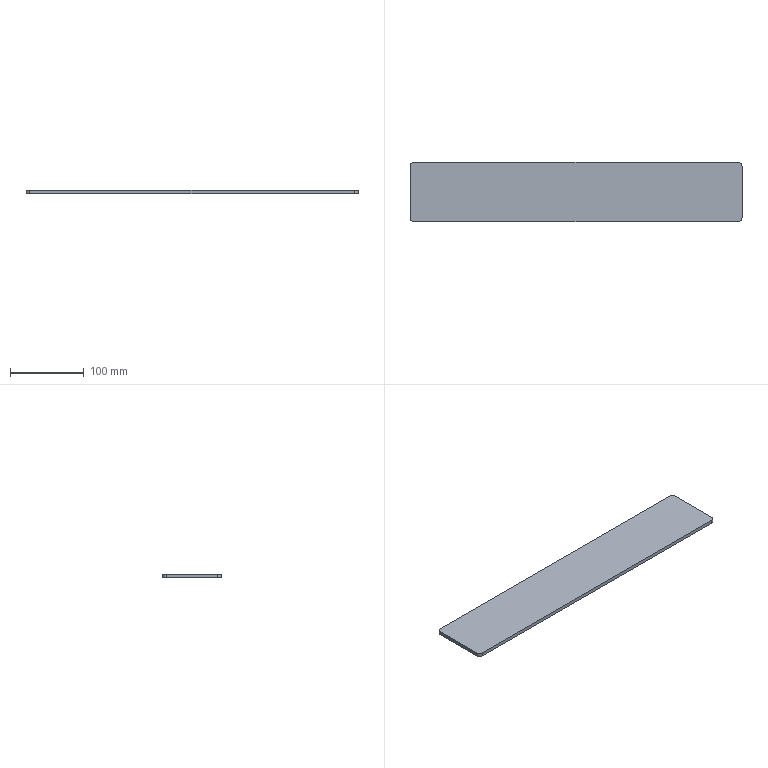Component | SolidWorks | VerticalMovingRectangularTubeWeldment-1_RectangularTubeWeldPlate2-1 | 1 solid | 10 faces | box 450 x 80 x 5 mm | volume 179893 mm3 | plane 6 | cylinder 4 | commonest cylinder face diameters 10 x4 | material Plain Carbon Steel
STEP:
#1=CARTESIAN_POINT('',(-0.9843,1.378,13.78));
#2=VERTEX_POINT('',#1);
#3=CARTESIAN_POINT('',(-0.9843,1.378,13.976));
#4=VERTEX_POINT('',#3);
#5=CARTESIAN_POINT('',(-0.9843,1.378,14.094));
#6=DIRECTION('',(0.,0.,1.));
#7=VECTOR('',#6,39.37);
#8=LINE('',#5,#7);
#9=EDGE_CURVE('',#2,#4,#8,.T.);
#10=ORIENTED_EDGE('',*,*,#9,.T.);
#11=CARTESIAN_POINT('',(-0.9843,-1.378,13.976));
#12=VERTEX_POINT('',#11);
#13=CARTESIAN_POINT('',(-0.9843,-1.575,13.976));
#14=DIRECTION('',(0.,-1.,0.));
#15=VECTOR('',#14,39.37);
#16=LINE('',#13,#15);
#17=EDGE_CURVE('',#4,#12,#16,.T.);
#18=ORIENTED_EDGE('',*,*,#17,.T.);
#19=CARTESIAN_POINT('',(-0.9843,-1.378,13.78));
#20=VERTEX_POINT('',#19);
#21=CARTESIAN_POINT('',(-0.9843,-1.378,14.094));
#22=DIRECTION('',(0.,0.,-1.));
#23=VECTOR('',#22,39.37);
#24=LINE('',#21,#23);
#25=EDGE_CURVE('',#12,#20,#24,.T.);
#26=ORIENTED_EDGE('',*,*,#25,.T.);
#27=CARTESIAN_POINT('',(-0.9843,-1.575,13.78));
#28=DIRECTION('',(0.,1.,0.));
#29=VECTOR('',#28,39.37);
#30=LINE('',#27,#29);
#31=EDGE_CURVE('',#20,#2,#30,.T.);
#32=ORIENTED_EDGE('',*,*,#31,.T.);
#33=EDGE_LOOP('',(#10,#18,#26,#32));
#34=FACE_OUTER_BOUND('',#33,.T.);
#35=CARTESIAN_POINT('',(-0.9843,-1.575,14.094));
#36=DIRECTION('',(-1.,0.,0.));
#37=DIRECTION('',(0.,-1.,0.));
#38=AXIS2_PLACEMENT_3D('',#35,#36,#37);
#39=PLANE('',#38);
#40=ADVANCED_FACE('',(#34),#39,.F.);
#41=CARTESIAN_POINT('',(-18.504,1.575,13.78));
#42=VERTEX_POINT('',#41);
#43=CARTESIAN_POINT('',(-18.504,1.575,13.976));
#44=VERTEX_POINT('',#43);
#45=CARTESIAN_POINT('',(-18.504,1.575,14.094));
#46=DIRECTION('',(0.,0.,1.));
#47=VECTOR('',#46,39.37);
#48=LINE('',#45,#47);
#49=EDGE_CURVE('',#42,#44,#48,.T.);
#50=ORIENTED_EDGE('',*,*,#49,.T.);
#51=CARTESIAN_POINT('',(-1.181,1.575,13.976));
#52=VERTEX_POINT('',#51);
#53=CARTESIAN_POINT('',(-18.701,1.575,13.976));
#54=DIRECTION('',(1.,0.,0.));
#55=VECTOR('',#54,39.37);
#56=LINE('',#53,#55);
#57=EDGE_CURVE('',#44,#52,#56,.T.);
#58=ORIENTED_EDGE('',*,*,#57,.T.);
#59=CARTESIAN_POINT('',(-1.181,1.575,13.78));
#60=VERTEX_POINT('',#59);
#61=CARTESIAN_POINT('',(-1.181,1.575,14.094));
#62=DIRECTION('',(0.,0.,-1.));
#63=VECTOR('',#62,39.37);
#64=LINE('',#61,#63);
#65=EDGE_CURVE('',#52,#60,#64,.T.);
#66=ORIENTED_EDGE('',*,*,#65,.T.);
#67=CARTESIAN_POINT('',(-18.701,1.575,13.78));
#68=DIRECTION('',(-1.,0.,0.));
#69=VECTOR('',#68,39.37);
#70=LINE('',#67,#69);
#71=EDGE_CURVE('',#60,#42,#70,.T.);
#72=ORIENTED_EDGE('',*,*,#71,.T.);
#73=EDGE_LOOP('',(#50,#58,#66,#72));
#74=FACE_OUTER_BOUND('',#73,.T.);
#75=CARTESIAN_POINT('',(-18.701,1.575,14.094));
#76=DIRECTION('',(0.,-1.,0.));
#77=DIRECTION('',(1.,0.,0.));
#78=AXIS2_PLACEMENT_3D('',#75,#76,#77);
#79=PLANE('',#78);
#80=ADVANCED_FACE('',(#74),#79,.F.);
#81=CARTESIAN_POINT('',(-18.701,-1.378,13.78));
#82=VERTEX_POINT('',#81);
#83=CARTESIAN_POINT('',(-18.701,-1.378,13.976));
#84=VERTEX_POINT('',#83);
#85=CARTESIAN_POINT('',(-18.701,-1.378,14.094));
#86=DIRECTION('',(0.,0.,1.));
#87=VECTOR('',#86,39.37);
#88=LINE('',#85,#87);
#89=EDGE_CURVE('',#82,#84,#88,.T.);
#90=ORIENTED_EDGE('',*,*,#89,.T.);
#91=CARTESIAN_POINT('',(-18.701,1.378,13.976));
#92=VERTEX_POINT('',#91);
#93=CARTESIAN_POINT('',(-18.701,1.988,13.976));
#94=DIRECTION('',(0.,-1.,0.));
#95=VECTOR('',#94,39.37);
#96=LINE('',#93,#95);
#97=EDGE_CURVE('',#92,#84,#96,.T.);
#98=ORIENTED_EDGE('',*,*,#97,.F.);
#99=CARTESIAN_POINT('',(-18.701,1.378,13.78));
#100=VERTEX_POINT('',#99);
#101=CARTESIAN_POINT('',(-18.701,1.378,14.094));
#102=DIRECTION('',(0.,0.,-1.));
#103=VECTOR('',#102,39.37);
#104=LINE('',#101,#103);
#105=EDGE_CURVE('',#92,#100,#104,.T.);
#106=ORIENTED_EDGE('',*,*,#105,.T.);
#107=CARTESIAN_POINT('',(-18.701,-1.575,13.78));
#108=DIRECTION('',(0.,-1.,0.));
#109=VECTOR('',#108,39.37);
#110=LINE('',#107,#109);
#111=EDGE_CURVE('',#100,#82,#110,.T.);
#112=ORIENTED_EDGE('',*,*,#111,.T.);
#113=EDGE_LOOP('',(#90,#98,#106,#112));
#114=FACE_OUTER_BOUND('',#113,.T.);
#115=CARTESIAN_POINT('',(-18.701,-1.575,14.094));
#116=DIRECTION('',(1.,0.,0.));
#117=DIRECTION('',(0.,1.,0.));
#118=AXIS2_PLACEMENT_3D('',#115,#116,#117);
#119=PLANE('',#118);
#120=ADVANCED_FACE('',(#114),#119,.F.);
#121=CARTESIAN_POINT('',(-1.181,-1.575,13.78));
#122=VERTEX_POINT('',#121);
#123=CARTESIAN_POINT('',(-1.181,-1.575,13.976));
#124=VERTEX_POINT('',#123);
#125=CARTESIAN_POINT('',(-1.181,-1.575,14.094));
#126=DIRECTION('',(0.,0.,1.));
#127=VECTOR('',#126,39.37);
#128=LINE('',#125,#127);
#129=EDGE_CURVE('',#122,#124,#128,.T.);
#130=ORIENTED_EDGE('',*,*,#129,.T.);
#131=CARTESIAN_POINT('',(-18.504,-1.575,13.976));
#132=VERTEX_POINT('',#131);
#133=CARTESIAN_POINT('',(-18.701,-1.575,13.976));
#134=DIRECTION('',(-1.,0.,0.));
#135=VECTOR('',#134,39.37);
#136=LINE('',#133,#135);
#137=EDGE_CURVE('',#124,#132,#136,.T.);
#138=ORIENTED_EDGE('',*,*,#137,.T.);
#139=CARTESIAN_POINT('',(-18.504,-1.575,13.78));
#140=VERTEX_POINT('',#139);
#141=CARTESIAN_POINT('',(-18.504,-1.575,14.094));
#142=DIRECTION('',(0.,0.,-1.));
#143=VECTOR('',#142,39.37);
#144=LINE('',#141,#143);
#145=EDGE_CURVE('',#132,#140,#144,.T.);
#146=ORIENTED_EDGE('',*,*,#145,.T.);
#147=CARTESIAN_POINT('',(-18.701,-1.575,13.78));
#148=DIRECTION('',(1.,0.,0.));
#149=VECTOR('',#148,39.37);
#150=LINE('',#147,#149);
#151=EDGE_CURVE('',#140,#122,#150,.T.);
#152=ORIENTED_EDGE('',*,*,#151,.T.);
#153=EDGE_LOOP('',(#130,#138,#146,#152));
#154=FACE_OUTER_BOUND('',#153,.T.);
#155=CARTESIAN_POINT('',(-18.701,-1.575,14.094));
#156=DIRECTION('',(0.,1.,0.));
#157=DIRECTION('',(-1.,0.,0.));
#158=AXIS2_PLACEMENT_3D('',#155,#156,#157);
#159=PLANE('',#158);
#160=ADVANCED_FACE('',(#154),#159,.F.);
#161=ORIENTED_EDGE('',*,*,#71,.F.);
#162=CARTESIAN_POINT('',(-1.181,1.378,13.78));
#163=DIRECTION('',(0.,0.,-1.));
#164=DIRECTION('',(0.,1.,0.));
#165=AXIS2_PLACEMENT_3D('',#162,#163,#164);
#166=CIRCLE('',#165,0.1969);
#167=EDGE_CURVE('',#60,#2,#166,.T.);
#168=ORIENTED_EDGE('',*,*,#167,.T.);
#169=ORIENTED_EDGE('',*,*,#31,.F.);
#170=CARTESIAN_POINT('',(-1.181,-1.378,13.78));
#171=DIRECTION('',(0.,0.,-1.));
#172=DIRECTION('',(0.,1.,0.));
#173=AXIS2_PLACEMENT_3D('',#170,#171,#172);
#174=CIRCLE('',#173,0.1969);
#175=EDGE_CURVE('',#20,#122,#174,.T.);
#176=ORIENTED_EDGE('',*,*,#175,.T.);
#177=ORIENTED_EDGE('',*,*,#151,.F.);
#178=CARTESIAN_POINT('',(-18.504,-1.378,13.78));
#179=DIRECTION('',(0.,0.,-1.));
#180=DIRECTION('',(0.,1.,0.));
#181=AXIS2_PLACEMENT_3D('',#178,#179,#180);
#182=CIRCLE('',#181,0.1969);
#183=EDGE_CURVE('',#140,#82,#182,.T.);
#184=ORIENTED_EDGE('',*,*,#183,.T.);
#185=ORIENTED_EDGE('',*,*,#111,.F.);
#186=CARTESIAN_POINT('',(-18.504,1.378,13.78));
#187=DIRECTION('',(0.,0.,-1.));
#188=DIRECTION('',(0.,1.,0.));
#189=AXIS2_PLACEMENT_3D('',#186,#187,#188);
#190=CIRCLE('',#189,0.1969);
#191=EDGE_CURVE('',#100,#42,#190,.T.);
#192=ORIENTED_EDGE('',*,*,#191,.T.);
#193=EDGE_LOOP('',(#161,#168,#169,#176,#177,#184,#185,#192));
#194=FACE_OUTER_BOUND('',#193,.T.);
#195=CARTESIAN_POINT('',(-9.843,0.,13.78));
#196=DIRECTION('',(0.,0.,-1.));
#197=DIRECTION('',(0.,1.,0.));
#198=AXIS2_PLACEMENT_3D('',#195,#196,#197);
#199=PLANE('',#198);
#200=ADVANCED_FACE('',(#194),#199,.T.);
#201=CARTESIAN_POINT('',(-1.181,1.378,13.976));
#202=DIRECTION('',(0.,0.,1.));
#203=DIRECTION('',(0.,1.,0.));
#204=AXIS2_PLACEMENT_3D('',#201,#202,#203);
#205=CIRCLE('',#204,0.1969);
#206=EDGE_CURVE('',#4,#52,#205,.T.);
#207=ORIENTED_EDGE('',*,*,#206,.F.);
#208=ORIENTED_EDGE('',*,*,#9,.F.);
#209=ORIENTED_EDGE('',*,*,#167,.F.);
#210=ORIENTED_EDGE('',*,*,#65,.F.);
#211=EDGE_LOOP('',(#207,#208,#209,#210));
#212=FACE_OUTER_BOUND('',#211,.T.);
#213=CARTESIAN_POINT('',(-1.181,1.378,14.094));
#214=DIRECTION('',(0.,0.,-1.));
#215=DIRECTION('',(0.,1.,0.));
#216=AXIS2_PLACEMENT_3D('',#213,#214,#215);
#217=CYLINDRICAL_SURFACE('',#216,0.1969);
#218=ADVANCED_FACE('',(#212),#217,.T.);
#219=CARTESIAN_POINT('',(-1.181,-1.378,13.976));
#220=DIRECTION('',(0.,0.,1.));
#221=DIRECTION('',(0.,1.,0.));
#222=AXIS2_PLACEMENT_3D('',#219,#220,#221);
#223=CIRCLE('',#222,0.1969);
#224=EDGE_CURVE('',#124,#12,#223,.T.);
#225=ORIENTED_EDGE('',*,*,#224,.F.);
#226=ORIENTED_EDGE('',*,*,#129,.F.);
#227=ORIENTED_EDGE('',*,*,#175,.F.);
#228=ORIENTED_EDGE('',*,*,#25,.F.);
#229=EDGE_LOOP('',(#225,#226,#227,#228));
#230=FACE_OUTER_BOUND('',#229,.T.);
#231=CARTESIAN_POINT('',(-1.181,-1.378,14.094));
#232=DIRECTION('',(0.,0.,-1.));
#233=DIRECTION('',(0.,1.,0.));
#234=AXIS2_PLACEMENT_3D('',#231,#232,#233);
#235=CYLINDRICAL_SURFACE('',#234,0.1969);
#236=ADVANCED_FACE('',(#230),#235,.T.);
#237=CARTESIAN_POINT('',(-18.504,-1.378,13.976));
#238=DIRECTION('',(0.,0.,1.));
#239=DIRECTION('',(0.,1.,0.));
#240=AXIS2_PLACEMENT_3D('',#237,#238,#239);
#241=CIRCLE('',#240,0.1969);
#242=EDGE_CURVE('',#84,#132,#241,.T.);
#243=ORIENTED_EDGE('',*,*,#242,.F.);
#244=ORIENTED_EDGE('',*,*,#89,.F.);
#245=ORIENTED_EDGE('',*,*,#183,.F.);
#246=ORIENTED_EDGE('',*,*,#145,.F.);
#247=EDGE_LOOP('',(#243,#244,#245,#246));
#248=FACE_OUTER_BOUND('',#247,.T.);
#249=CARTESIAN_POINT('',(-18.504,-1.378,14.094));
#250=DIRECTION('',(0.,0.,-1.));
#251=DIRECTION('',(0.,1.,0.));
#252=AXIS2_PLACEMENT_3D('',#249,#250,#251);
#253=CYLINDRICAL_SURFACE('',#252,0.1969);
#254=ADVANCED_FACE('',(#248),#253,.T.);
#255=CARTESIAN_POINT('',(-18.504,1.378,13.976));
#256=DIRECTION('',(0.,0.,1.));
#257=DIRECTION('',(0.,1.,0.));
#258=AXIS2_PLACEMENT_3D('',#255,#256,#257);
#259=CIRCLE('',#258,0.1969);
#260=EDGE_CURVE('',#44,#92,#259,.T.);
#261=ORIENTED_EDGE('',*,*,#260,.F.);
#262=ORIENTED_EDGE('',*,*,#49,.F.);
#263=ORIENTED_EDGE('',*,*,#191,.F.);
#264=ORIENTED_EDGE('',*,*,#105,.F.);
#265=EDGE_LOOP('',(#261,#262,#263,#264));
#266=FACE_OUTER_BOUND('',#265,.T.);
#267=CARTESIAN_POINT('',(-18.504,1.378,14.094));
#268=DIRECTION('',(0.,0.,-1.));
#269=DIRECTION('',(0.,1.,0.));
#270=AXIS2_PLACEMENT_3D('',#267,#268,#269);
#271=CYLINDRICAL_SURFACE('',#270,0.1969);
#272=ADVANCED_FACE('',(#266),#271,.T.);
#273=ORIENTED_EDGE('',*,*,#242,.T.);
#274=ORIENTED_EDGE('',*,*,#137,.F.);
#275=ORIENTED_EDGE('',*,*,#224,.T.);
#276=ORIENTED_EDGE('',*,*,#17,.F.);
#277=ORIENTED_EDGE('',*,*,#206,.T.);
#278=ORIENTED_EDGE('',*,*,#57,.F.);
#279=ORIENTED_EDGE('',*,*,#260,.T.);
#280=ORIENTED_EDGE('',*,*,#97,.T.);
#281=EDGE_LOOP('',(#273,#274,#275,#276,#277,#278,#279,#280));
#282=FACE_OUTER_BOUND('',#281,.T.);
#283=CARTESIAN_POINT('',(20.079,1.988,13.976));
#284=DIRECTION('',(0.,0.,-1.));
#285=DIRECTION('',(-1.,0.,0.));
#286=AXIS2_PLACEMENT_3D('',#283,#284,#285);
#287=PLANE('',#286);
#288=ADVANCED_FACE('',(#282),#287,.F.);
#289=CLOSED_SHELL('',(#40,#80,#120,#160,#200,#218,#236,#254,#272,#288));
#290=MANIFOLD_SOLID_BREP('',#289);
#291=CARTESIAN_POINT('',(0.,0.,0.));
#292=DIRECTION('',(0.,0.,1.));
#293=DIRECTION('',(1.,0.,0.));
#294=AXIS2_PLACEMENT_3D('',#291,#292,#293);
#295=(LENGTH_UNIT()NAMED_UNIT(*)SI_UNIT($,.METRE.));
#296=LENGTH_MEASURE_WITH_UNIT(LENGTH_MEASURE(0.0254),#295);
#297=DIMENSIONAL_EXPONENTS(1.,0.,0.,0.,0.,0.,0.);
#298=(CONVERSION_BASED_UNIT('',#296)LENGTH_UNIT()NAMED_UNIT(#297));
#299=UNCERTAINTY_MEASURE_WITH_UNIT(LENGTH_MEASURE(0.00001),#298,'','');
#300=(NAMED_UNIT(*)PLANE_ANGLE_UNIT()SI_UNIT($,.RADIAN.));
#301=(NAMED_UNIT(*)SI_UNIT($,.STERADIAN.)SOLID_ANGLE_UNIT());
#302=(GEOMETRIC_REPRESENTATION_CONTEXT(3)GLOBAL_UNCERTAINTY_ASSIGNED_CONTEXT((#299))GLOBAL_UNIT_ASSIGNED_CONTEXT((#298,#300,#301))REPRESENTATION_CONTEXT('',''));
#303=ADVANCED_BREP_SHAPE_REPRESENTATION('',(#290,#294),#302);
#304=COLOUR_RGB('',0.7922,0.8196,0.9333);
#305=FILL_AREA_STYLE_COLOUR('',#304);
#306=FILL_AREA_STYLE('',(#305));
#307=SURFACE_STYLE_FILL_AREA(#306);
#308=SURFACE_SIDE_STYLE('',(#307));
#309=SURFACE_STYLE_USAGE(.BOTH.,#308);
#310=PRESENTATION_STYLE_ASSIGNMENT((#309));
#311=STYLED_ITEM('',(#310),#290);
#312=(LENGTH_UNIT()NAMED_UNIT(*)SI_UNIT($,.METRE.));
#313=LENGTH_MEASURE_WITH_UNIT(LENGTH_MEASURE(0.0254),#312);
#314=DIMENSIONAL_EXPONENTS(1.,0.,0.,0.,0.,0.,0.);
#315=(CONVERSION_BASED_UNIT('',#313)LENGTH_UNIT()NAMED_UNIT(#314));
#316=UNCERTAINTY_MEASURE_WITH_UNIT(LENGTH_MEASURE(0.00001),#315,'','');
#317=(NAMED_UNIT(*)PLANE_ANGLE_UNIT()SI_UNIT($,.RADIAN.));
#318=(NAMED_UNIT(*)SI_UNIT($,.STERADIAN.)SOLID_ANGLE_UNIT());
#319=(GEOMETRIC_REPRESENTATION_CONTEXT(3)GLOBAL_UNCERTAINTY_ASSIGNED_CONTEXT((#316))GLOBAL_UNIT_ASSIGNED_CONTEXT((#315,#317,#318))REPRESENTATION_CONTEXT('',''));
#320=MECHANICAL_DESIGN_GEOMETRIC_PRESENTATION_REPRESENTATION('',(#311),#319);
#321=PRESENTATION_LAYER_ASSIGNMENT('','',(#311));